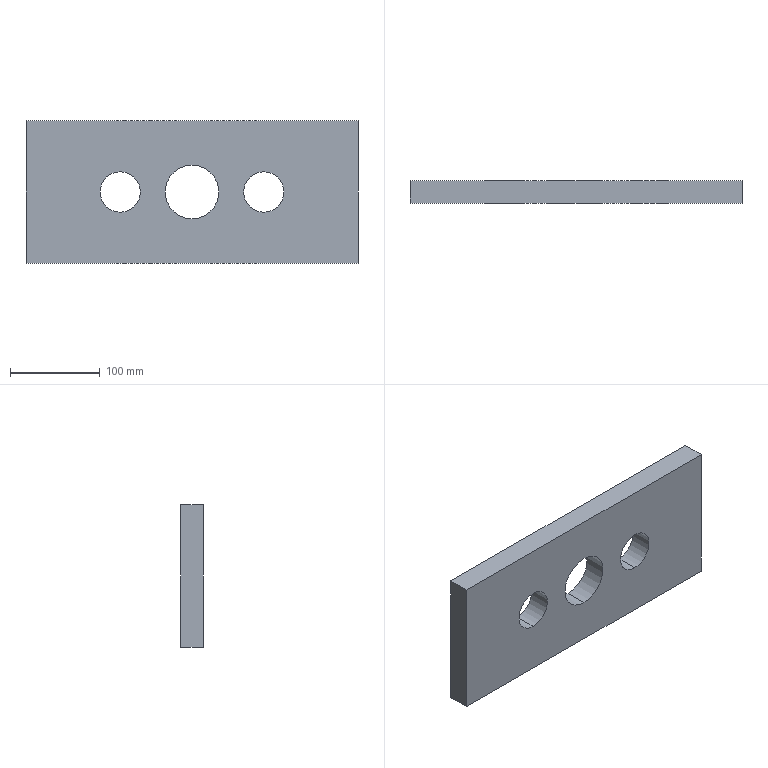Component | SolidWorks | NitrogenSupportUpperPlate-331MachineTool-1 | 1 solid | 12 faces | box 370 x 25 x 159 mm | volume 1320543 mm3 | cylinder 6 | plane 6 | commonest cylinder face diameters 45 x4 60 x2
STEP:
#1=COLOUR_RGB('',0.7922,0.8196,0.9333);
#2=FILL_AREA_STYLE_COLOUR('',#1);
#3=FILL_AREA_STYLE('',(#2));
#4=SURFACE_STYLE_FILL_AREA(#3);
#5=SURFACE_SIDE_STYLE('',(#4));
#6=SURFACE_STYLE_USAGE(.BOTH.,#5);
#7=PRESENTATION_STYLE_ASSIGNMENT((#6));
#8=CARTESIAN_POINT('',(-4.003,32.616,28.099));
#9=VERTEX_POINT('',#8);
#10=CARTESIAN_POINT('',(-4.003,32.616,25.737));
#11=VERTEX_POINT('',#10);
#12=CARTESIAN_POINT('',(-4.003,32.616,26.918));
#13=DIRECTION('',(0.,-1.,0.));
#14=DIRECTION('',(0.,0.,-1.));
#15=AXIS2_PLACEMENT_3D('',#12,#13,#14);
#16=CIRCLE('',#15,1.181);
#17=EDGE_CURVE('',#9,#11,#16,.T.);
#18=ORIENTED_EDGE('',*,*,#17,.F.);
#19=CARTESIAN_POINT('',(-4.003,31.631,28.099));
#20=VERTEX_POINT('',#19);
#21=CARTESIAN_POINT('',(-4.003,32.616,28.099));
#22=DIRECTION('',(0.,-1.,0.));
#23=VECTOR('',#22,39.37);
#24=LINE('',#21,#23);
#25=EDGE_CURVE('',#9,#20,#24,.T.);
#26=ORIENTED_EDGE('',*,*,#25,.T.);
#27=CARTESIAN_POINT('',(-4.003,31.631,25.737));
#28=VERTEX_POINT('',#27);
#29=CARTESIAN_POINT('',(-4.003,31.631,26.918));
#30=DIRECTION('',(0.,-1.,0.));
#31=DIRECTION('',(0.,0.,-1.));
#32=AXIS2_PLACEMENT_3D('',#29,#30,#31);
#33=CIRCLE('',#32,1.181);
#34=EDGE_CURVE('',#20,#28,#33,.T.);
#35=ORIENTED_EDGE('',*,*,#34,.T.);
#36=CARTESIAN_POINT('',(-4.003,32.616,25.737));
#37=DIRECTION('',(0.,-1.,0.));
#38=VECTOR('',#37,39.37);
#39=LINE('',#36,#38);
#40=EDGE_CURVE('',#11,#28,#39,.T.);
#41=ORIENTED_EDGE('',*,*,#40,.F.);
#42=EDGE_LOOP('',(#18,#26,#35,#41));
#43=FACE_OUTER_BOUND('',#42,.T.);
#44=CARTESIAN_POINT('',(-4.003,32.616,26.918));
#45=DIRECTION('',(0.,-1.,0.));
#46=DIRECTION('',(0.,0.,-1.));
#47=AXIS2_PLACEMENT_3D('',#44,#45,#46);
#48=CYLINDRICAL_SURFACE('',#47,1.181);
#49=ADVANCED_FACE('',(#43),#48,.F.);
#50=CARTESIAN_POINT('',(-7.153,32.616,27.804));
#51=VERTEX_POINT('',#50);
#52=CARTESIAN_POINT('',(-7.153,32.616,26.032));
#53=VERTEX_POINT('',#52);
#54=CARTESIAN_POINT('',(-7.153,32.616,26.918));
#55=DIRECTION('',(0.,-1.,0.));
#56=DIRECTION('',(0.,0.,-1.));
#57=AXIS2_PLACEMENT_3D('',#54,#55,#56);
#58=CIRCLE('',#57,0.8858);
#59=EDGE_CURVE('',#51,#53,#58,.T.);
#60=ORIENTED_EDGE('',*,*,#59,.F.);
#61=CARTESIAN_POINT('',(-7.153,31.631,27.804));
#62=VERTEX_POINT('',#61);
#63=CARTESIAN_POINT('',(-7.153,32.616,27.804));
#64=DIRECTION('',(0.,-1.,0.));
#65=VECTOR('',#64,39.37);
#66=LINE('',#63,#65);
#67=EDGE_CURVE('',#51,#62,#66,.T.);
#68=ORIENTED_EDGE('',*,*,#67,.T.);
#69=CARTESIAN_POINT('',(-7.153,31.631,26.032));
#70=VERTEX_POINT('',#69);
#71=CARTESIAN_POINT('',(-7.153,31.631,26.918));
#72=DIRECTION('',(0.,-1.,0.));
#73=DIRECTION('',(0.,0.,-1.));
#74=AXIS2_PLACEMENT_3D('',#71,#72,#73);
#75=CIRCLE('',#74,0.8858);
#76=EDGE_CURVE('',#62,#70,#75,.T.);
#77=ORIENTED_EDGE('',*,*,#76,.T.);
#78=CARTESIAN_POINT('',(-7.153,32.616,26.032));
#79=DIRECTION('',(0.,-1.,0.));
#80=VECTOR('',#79,39.37);
#81=LINE('',#78,#80);
#82=EDGE_CURVE('',#53,#70,#81,.T.);
#83=ORIENTED_EDGE('',*,*,#82,.F.);
#84=EDGE_LOOP('',(#60,#68,#77,#83));
#85=FACE_OUTER_BOUND('',#84,.T.);
#86=CARTESIAN_POINT('',(-7.153,32.616,26.918));
#87=DIRECTION('',(0.,-1.,0.));
#88=DIRECTION('',(0.,0.,-1.));
#89=AXIS2_PLACEMENT_3D('',#86,#87,#88);
#90=CYLINDRICAL_SURFACE('',#89,0.8858);
#91=ADVANCED_FACE('',(#85),#90,.F.);
#92=CARTESIAN_POINT('',(-0.8536,32.616,27.804));
#93=VERTEX_POINT('',#92);
#94=CARTESIAN_POINT('',(-0.8536,32.616,26.032));
#95=VERTEX_POINT('',#94);
#96=CARTESIAN_POINT('',(-0.8536,32.616,26.918));
#97=DIRECTION('',(0.,-1.,0.));
#98=DIRECTION('',(0.,0.,-1.));
#99=AXIS2_PLACEMENT_3D('',#96,#97,#98);
#100=CIRCLE('',#99,0.8858);
#101=EDGE_CURVE('',#93,#95,#100,.T.);
#102=ORIENTED_EDGE('',*,*,#101,.F.);
#103=CARTESIAN_POINT('',(-0.8536,31.631,27.804));
#104=VERTEX_POINT('',#103);
#105=CARTESIAN_POINT('',(-0.8536,32.616,27.804));
#106=DIRECTION('',(0.,-1.,0.));
#107=VECTOR('',#106,39.37);
#108=LINE('',#105,#107);
#109=EDGE_CURVE('',#93,#104,#108,.T.);
#110=ORIENTED_EDGE('',*,*,#109,.T.);
#111=CARTESIAN_POINT('',(-0.8536,31.631,26.032));
#112=VERTEX_POINT('',#111);
#113=CARTESIAN_POINT('',(-0.8536,31.631,26.918));
#114=DIRECTION('',(0.,-1.,0.));
#115=DIRECTION('',(0.,0.,-1.));
#116=AXIS2_PLACEMENT_3D('',#113,#114,#115);
#117=CIRCLE('',#116,0.8858);
#118=EDGE_CURVE('',#104,#112,#117,.T.);
#119=ORIENTED_EDGE('',*,*,#118,.T.);
#120=CARTESIAN_POINT('',(-0.8536,32.616,26.032));
#121=DIRECTION('',(0.,-1.,0.));
#122=VECTOR('',#121,39.37);
#123=LINE('',#120,#122);
#124=EDGE_CURVE('',#95,#112,#123,.T.);
#125=ORIENTED_EDGE('',*,*,#124,.F.);
#126=EDGE_LOOP('',(#102,#110,#119,#125));
#127=FACE_OUTER_BOUND('',#126,.T.);
#128=CARTESIAN_POINT('',(-0.8536,32.616,26.918));
#129=DIRECTION('',(0.,-1.,0.));
#130=DIRECTION('',(0.,0.,-1.));
#131=AXIS2_PLACEMENT_3D('',#128,#129,#130);
#132=CYLINDRICAL_SURFACE('',#131,0.8858);
#133=ADVANCED_FACE('',(#127),#132,.F.);
#134=CARTESIAN_POINT('',(-11.287,32.616,23.788));
#135=VERTEX_POINT('',#134);
#136=CARTESIAN_POINT('',(-11.287,32.616,30.048));
#137=VERTEX_POINT('',#136);
#138=CARTESIAN_POINT('',(-11.287,32.616,23.788));
#139=DIRECTION('',(0.,0.,1.));
#140=VECTOR('',#139,39.37);
#141=LINE('',#138,#140);
#142=EDGE_CURVE('',#135,#137,#141,.T.);
#143=ORIENTED_EDGE('',*,*,#142,.F.);
#144=CARTESIAN_POINT('',(-11.287,31.631,23.788));
#145=VERTEX_POINT('',#144);
#146=CARTESIAN_POINT('',(-11.287,31.631,23.788));
#147=DIRECTION('',(0.,1.,0.));
#148=VECTOR('',#147,39.37);
#149=LINE('',#146,#148);
#150=EDGE_CURVE('',#145,#135,#149,.T.);
#151=ORIENTED_EDGE('',*,*,#150,.F.);
#152=CARTESIAN_POINT('',(-11.287,31.631,30.048));
#153=VERTEX_POINT('',#152);
#154=CARTESIAN_POINT('',(-11.287,31.631,23.788));
#155=DIRECTION('',(0.,0.,1.));
#156=VECTOR('',#155,39.37);
#157=LINE('',#154,#156);
#158=EDGE_CURVE('',#145,#153,#157,.T.);
#159=ORIENTED_EDGE('',*,*,#158,.T.);
#160=CARTESIAN_POINT('',(-11.287,31.631,30.048));
#161=DIRECTION('',(0.,1.,0.));
#162=VECTOR('',#161,39.37);
#163=LINE('',#160,#162);
#164=EDGE_CURVE('',#153,#137,#163,.T.);
#165=ORIENTED_EDGE('',*,*,#164,.T.);
#166=EDGE_LOOP('',(#143,#151,#159,#165));
#167=FACE_OUTER_BOUND('',#166,.T.);
#168=CARTESIAN_POINT('',(-11.287,31.631,23.788));
#169=DIRECTION('',(-1.,0.,0.));
#170=DIRECTION('',(0.,0.,1.));
#171=AXIS2_PLACEMENT_3D('',#168,#169,#170);
#172=PLANE('',#171);
#173=ADVANCED_FACE('',(#167),#172,.T.);
#174=CARTESIAN_POINT('',(3.28,32.616,23.788));
#175=VERTEX_POINT('',#174);
#176=CARTESIAN_POINT('',(-11.287,32.616,23.788));
#177=DIRECTION('',(-1.,0.,0.));
#178=VECTOR('',#177,39.37);
#179=LINE('',#176,#178);
#180=EDGE_CURVE('',#175,#135,#179,.T.);
#181=ORIENTED_EDGE('',*,*,#180,.F.);
#182=CARTESIAN_POINT('',(3.28,31.631,23.788));
#183=VERTEX_POINT('',#182);
#184=CARTESIAN_POINT('',(3.28,31.631,23.788));
#185=DIRECTION('',(0.,1.,0.));
#186=VECTOR('',#185,39.37);
#187=LINE('',#184,#186);
#188=EDGE_CURVE('',#183,#175,#187,.T.);
#189=ORIENTED_EDGE('',*,*,#188,.F.);
#190=CARTESIAN_POINT('',(-11.287,31.631,23.788));
#191=DIRECTION('',(-1.,0.,0.));
#192=VECTOR('',#191,39.37);
#193=LINE('',#190,#192);
#194=EDGE_CURVE('',#183,#145,#193,.T.);
#195=ORIENTED_EDGE('',*,*,#194,.T.);
#196=ORIENTED_EDGE('',*,*,#150,.T.);
#197=EDGE_LOOP('',(#181,#189,#195,#196));
#198=FACE_OUTER_BOUND('',#197,.T.);
#199=CARTESIAN_POINT('',(-11.287,31.631,23.788));
#200=DIRECTION('',(0.,0.,-1.));
#201=DIRECTION('',(-1.,0.,0.));
#202=AXIS2_PLACEMENT_3D('',#199,#200,#201);
#203=PLANE('',#202);
#204=ADVANCED_FACE('',(#198),#203,.T.);
#205=CARTESIAN_POINT('',(3.28,32.616,30.048));
#206=VERTEX_POINT('',#205);
#207=CARTESIAN_POINT('',(3.28,32.616,23.788));
#208=DIRECTION('',(0.,0.,-1.));
#209=VECTOR('',#208,39.37);
#210=LINE('',#207,#209);
#211=EDGE_CURVE('',#206,#175,#210,.T.);
#212=ORIENTED_EDGE('',*,*,#211,.F.);
#213=CARTESIAN_POINT('',(3.28,31.631,30.048));
#214=VERTEX_POINT('',#213);
#215=CARTESIAN_POINT('',(3.28,31.631,30.048));
#216=DIRECTION('',(0.,1.,0.));
#217=VECTOR('',#216,39.37);
#218=LINE('',#215,#217);
#219=EDGE_CURVE('',#214,#206,#218,.T.);
#220=ORIENTED_EDGE('',*,*,#219,.F.);
#221=CARTESIAN_POINT('',(3.28,31.631,23.788));
#222=DIRECTION('',(0.,0.,-1.));
#223=VECTOR('',#222,39.37);
#224=LINE('',#221,#223);
#225=EDGE_CURVE('',#214,#183,#224,.T.);
#226=ORIENTED_EDGE('',*,*,#225,.T.);
#227=ORIENTED_EDGE('',*,*,#188,.T.);
#228=EDGE_LOOP('',(#212,#220,#226,#227));
#229=FACE_OUTER_BOUND('',#228,.T.);
#230=CARTESIAN_POINT('',(3.28,31.631,23.788));
#231=DIRECTION('',(1.,0.,0.));
#232=DIRECTION('',(0.,0.,-1.));
#233=AXIS2_PLACEMENT_3D('',#230,#231,#232);
#234=PLANE('',#233);
#235=ADVANCED_FACE('',(#229),#234,.T.);
#236=CARTESIAN_POINT('',(-11.287,32.616,30.048));
#237=DIRECTION('',(1.,0.,0.));
#238=VECTOR('',#237,39.37);
#239=LINE('',#236,#238);
#240=EDGE_CURVE('',#137,#206,#239,.T.);
#241=ORIENTED_EDGE('',*,*,#240,.F.);
#242=ORIENTED_EDGE('',*,*,#164,.F.);
#243=CARTESIAN_POINT('',(-11.287,31.631,30.048));
#244=DIRECTION('',(1.,0.,0.));
#245=VECTOR('',#244,39.37);
#246=LINE('',#243,#245);
#247=EDGE_CURVE('',#153,#214,#246,.T.);
#248=ORIENTED_EDGE('',*,*,#247,.T.);
#249=ORIENTED_EDGE('',*,*,#219,.T.);
#250=EDGE_LOOP('',(#241,#242,#248,#249));
#251=FACE_OUTER_BOUND('',#250,.T.);
#252=CARTESIAN_POINT('',(-11.287,31.631,30.048));
#253=DIRECTION('',(0.,0.,1.));
#254=DIRECTION('',(1.,0.,0.));
#255=AXIS2_PLACEMENT_3D('',#252,#253,#254);
#256=PLANE('',#255);
#257=ADVANCED_FACE('',(#251),#256,.T.);
#258=CARTESIAN_POINT('',(-4.003,31.631,26.918));
#259=DIRECTION('',(0.,-1.,0.));
#260=DIRECTION('',(0.,0.,-1.));
#261=AXIS2_PLACEMENT_3D('',#258,#259,#260);
#262=CIRCLE('',#261,1.181);
#263=EDGE_CURVE('',#28,#20,#262,.T.);
#264=ORIENTED_EDGE('',*,*,#263,.F.);
#265=ORIENTED_EDGE('',*,*,#34,.F.);
#266=EDGE_LOOP('',(#264,#265));
#267=FACE_BOUND('',#266,.T.);
#268=CARTESIAN_POINT('',(-7.153,31.631,26.918));
#269=DIRECTION('',(0.,-1.,0.));
#270=DIRECTION('',(0.,0.,-1.));
#271=AXIS2_PLACEMENT_3D('',#268,#269,#270);
#272=CIRCLE('',#271,0.8858);
#273=EDGE_CURVE('',#70,#62,#272,.T.);
#274=ORIENTED_EDGE('',*,*,#273,.F.);
#275=ORIENTED_EDGE('',*,*,#76,.F.);
#276=EDGE_LOOP('',(#274,#275));
#277=FACE_BOUND('',#276,.T.);
#278=CARTESIAN_POINT('',(-0.8536,31.631,26.918));
#279=DIRECTION('',(0.,-1.,0.));
#280=DIRECTION('',(0.,0.,-1.));
#281=AXIS2_PLACEMENT_3D('',#278,#279,#280);
#282=CIRCLE('',#281,0.8858);
#283=EDGE_CURVE('',#112,#104,#282,.T.);
#284=ORIENTED_EDGE('',*,*,#283,.F.);
#285=ORIENTED_EDGE('',*,*,#118,.F.);
#286=EDGE_LOOP('',(#284,#285));
#287=FACE_BOUND('',#286,.T.);
#288=ORIENTED_EDGE('',*,*,#158,.F.);
#289=ORIENTED_EDGE('',*,*,#194,.F.);
#290=ORIENTED_EDGE('',*,*,#225,.F.);
#291=ORIENTED_EDGE('',*,*,#247,.F.);
#292=EDGE_LOOP('',(#288,#289,#290,#291));
#293=FACE_OUTER_BOUND('',#292,.T.);
#294=CARTESIAN_POINT('',(-3.782,31.631,24.912));
#295=DIRECTION('',(0.,1.,0.));
#296=DIRECTION('',(0.,0.,1.));
#297=AXIS2_PLACEMENT_3D('',#294,#295,#296);
#298=PLANE('',#297);
#299=ADVANCED_FACE('',(#267,#277,#287,#293),#298,.F.);
#300=CARTESIAN_POINT('',(-4.003,32.616,26.918));
#301=DIRECTION('',(0.,-1.,0.));
#302=DIRECTION('',(0.,0.,-1.));
#303=AXIS2_PLACEMENT_3D('',#300,#301,#302);
#304=CIRCLE('',#303,1.181);
#305=EDGE_CURVE('',#11,#9,#304,.T.);
#306=ORIENTED_EDGE('',*,*,#305,.T.);
#307=ORIENTED_EDGE('',*,*,#17,.T.);
#308=EDGE_LOOP('',(#306,#307));
#309=FACE_BOUND('',#308,.T.);
#310=CARTESIAN_POINT('',(-7.153,32.616,26.918));
#311=DIRECTION('',(0.,-1.,0.));
#312=DIRECTION('',(0.,0.,-1.));
#313=AXIS2_PLACEMENT_3D('',#310,#311,#312);
#314=CIRCLE('',#313,0.8858);
#315=EDGE_CURVE('',#53,#51,#314,.T.);
#316=ORIENTED_EDGE('',*,*,#315,.T.);
#317=ORIENTED_EDGE('',*,*,#59,.T.);
#318=EDGE_LOOP('',(#316,#317));
#319=FACE_BOUND('',#318,.T.);
#320=CARTESIAN_POINT('',(-0.8536,32.616,26.918));
#321=DIRECTION('',(0.,-1.,0.));
#322=DIRECTION('',(0.,0.,-1.));
#323=AXIS2_PLACEMENT_3D('',#320,#321,#322);
#324=CIRCLE('',#323,0.8858);
#325=EDGE_CURVE('',#95,#93,#324,.T.);
#326=ORIENTED_EDGE('',*,*,#325,.T.);
#327=ORIENTED_EDGE('',*,*,#101,.T.);
#328=EDGE_LOOP('',(#326,#327));
#329=FACE_BOUND('',#328,.T.);
#330=ORIENTED_EDGE('',*,*,#142,.T.);
#331=ORIENTED_EDGE('',*,*,#240,.T.);
#332=ORIENTED_EDGE('',*,*,#211,.T.);
#333=ORIENTED_EDGE('',*,*,#180,.T.);
#334=EDGE_LOOP('',(#330,#331,#332,#333));
#335=FACE_OUTER_BOUND('',#334,.T.);
#336=CARTESIAN_POINT('',(-3.782,32.616,24.912));
#337=DIRECTION('',(0.,1.,0.));
#338=DIRECTION('',(0.,0.,1.));
#339=AXIS2_PLACEMENT_3D('',#336,#337,#338);
#340=PLANE('',#339);
#341=ADVANCED_FACE('',(#309,#319,#329,#335),#340,.T.);
#342=ORIENTED_EDGE('',*,*,#109,.F.);
#343=ORIENTED_EDGE('',*,*,#325,.F.);
#344=ORIENTED_EDGE('',*,*,#124,.T.);
#345=ORIENTED_EDGE('',*,*,#283,.T.);
#346=EDGE_LOOP('',(#342,#343,#344,#345));
#347=FACE_OUTER_BOUND('',#346,.T.);
#348=CARTESIAN_POINT('',(-0.8536,32.616,26.918));
#349=DIRECTION('',(0.,-1.,0.));
#350=DIRECTION('',(0.,0.,-1.));
#351=AXIS2_PLACEMENT_3D('',#348,#349,#350);
#352=CYLINDRICAL_SURFACE('',#351,0.8858);
#353=ADVANCED_FACE('',(#347),#352,.F.);
#354=ORIENTED_EDGE('',*,*,#67,.F.);
#355=ORIENTED_EDGE('',*,*,#315,.F.);
#356=ORIENTED_EDGE('',*,*,#82,.T.);
#357=ORIENTED_EDGE('',*,*,#273,.T.);
#358=EDGE_LOOP('',(#354,#355,#356,#357));
#359=FACE_OUTER_BOUND('',#358,.T.);
#360=CARTESIAN_POINT('',(-7.153,32.616,26.918));
#361=DIRECTION('',(0.,-1.,0.));
#362=DIRECTION('',(0.,0.,-1.));
#363=AXIS2_PLACEMENT_3D('',#360,#361,#362);
#364=CYLINDRICAL_SURFACE('',#363,0.8858);
#365=ADVANCED_FACE('',(#359),#364,.F.);
#366=ORIENTED_EDGE('',*,*,#25,.F.);
#367=ORIENTED_EDGE('',*,*,#305,.F.);
#368=ORIENTED_EDGE('',*,*,#40,.T.);
#369=ORIENTED_EDGE('',*,*,#263,.T.);
#370=EDGE_LOOP('',(#366,#367,#368,#369));
#371=FACE_OUTER_BOUND('',#370,.T.);
#372=CARTESIAN_POINT('',(-4.003,32.616,26.918));
#373=DIRECTION('',(0.,-1.,0.));
#374=DIRECTION('',(0.,0.,-1.));
#375=AXIS2_PLACEMENT_3D('',#372,#373,#374);
#376=CYLINDRICAL_SURFACE('',#375,1.181);
#377=ADVANCED_FACE('',(#371),#376,.F.);
#378=CLOSED_SHELL('',(#49,#91,#133,#173,#204,#235,#257,#299,#341,#353,#365,#377));
#379=MANIFOLD_SOLID_BREP('',#378);
#380=STYLED_ITEM('',(#7),#379);
#381=(LENGTH_UNIT()NAMED_UNIT(*)SI_UNIT($,.METRE.));
#382=LENGTH_MEASURE_WITH_UNIT(LENGTH_MEASURE(0.0254),#381);
#383=DIMENSIONAL_EXPONENTS(1.,0.,0.,0.,0.,0.,0.);
#384=(CONVERSION_BASED_UNIT('',#382)LENGTH_UNIT()NAMED_UNIT(#383));
#385=UNCERTAINTY_MEASURE_WITH_UNIT(LENGTH_MEASURE(0.00001),#384,'','');
#386=(NAMED_UNIT(*)PLANE_ANGLE_UNIT()SI_UNIT($,.RADIAN.));
#387=(NAMED_UNIT(*)SI_UNIT($,.STERADIAN.)SOLID_ANGLE_UNIT());
#388=(GEOMETRIC_REPRESENTATION_CONTEXT(3)GLOBAL_UNCERTAINTY_ASSIGNED_CONTEXT((#385))GLOBAL_UNIT_ASSIGNED_CONTEXT((#384,#386,#387))REPRESENTATION_CONTEXT('',''));
#389=MECHANICAL_DESIGN_GEOMETRIC_PRESENTATION_REPRESENTATION('',(#380),#388);
#390=PRESENTATION_LAYER_ASSIGNMENT('','',(#380));
#391=CARTESIAN_POINT('',(0.,0.,0.));
#392=DIRECTION('',(0.,0.,1.));
#393=DIRECTION('',(1.,0.,0.));
#394=AXIS2_PLACEMENT_3D('',#391,#392,#393);
#395=(LENGTH_UNIT()NAMED_UNIT(*)SI_UNIT($,.METRE.));
#396=LENGTH_MEASURE_WITH_UNIT(LENGTH_MEASURE(0.0254),#395);
#397=DIMENSIONAL_EXPONENTS(1.,0.,0.,0.,0.,0.,0.);
#398=(CONVERSION_BASED_UNIT('',#396)LENGTH_UNIT()NAMED_UNIT(#397));
#399=UNCERTAINTY_MEASURE_WITH_UNIT(LENGTH_MEASURE(0.00001),#398,'','');
#400=(NAMED_UNIT(*)PLANE_ANGLE_UNIT()SI_UNIT($,.RADIAN.));
#401=(NAMED_UNIT(*)SI_UNIT($,.STERADIAN.)SOLID_ANGLE_UNIT());
#402=(GEOMETRIC_REPRESENTATION_CONTEXT(3)GLOBAL_UNCERTAINTY_ASSIGNED_CONTEXT((#399))GLOBAL_UNIT_ASSIGNED_CONTEXT((#398,#400,#401))REPRESENTATION_CONTEXT('',''));
#403=ADVANCED_BREP_SHAPE_REPRESENTATION('',(#379,#394),#402);